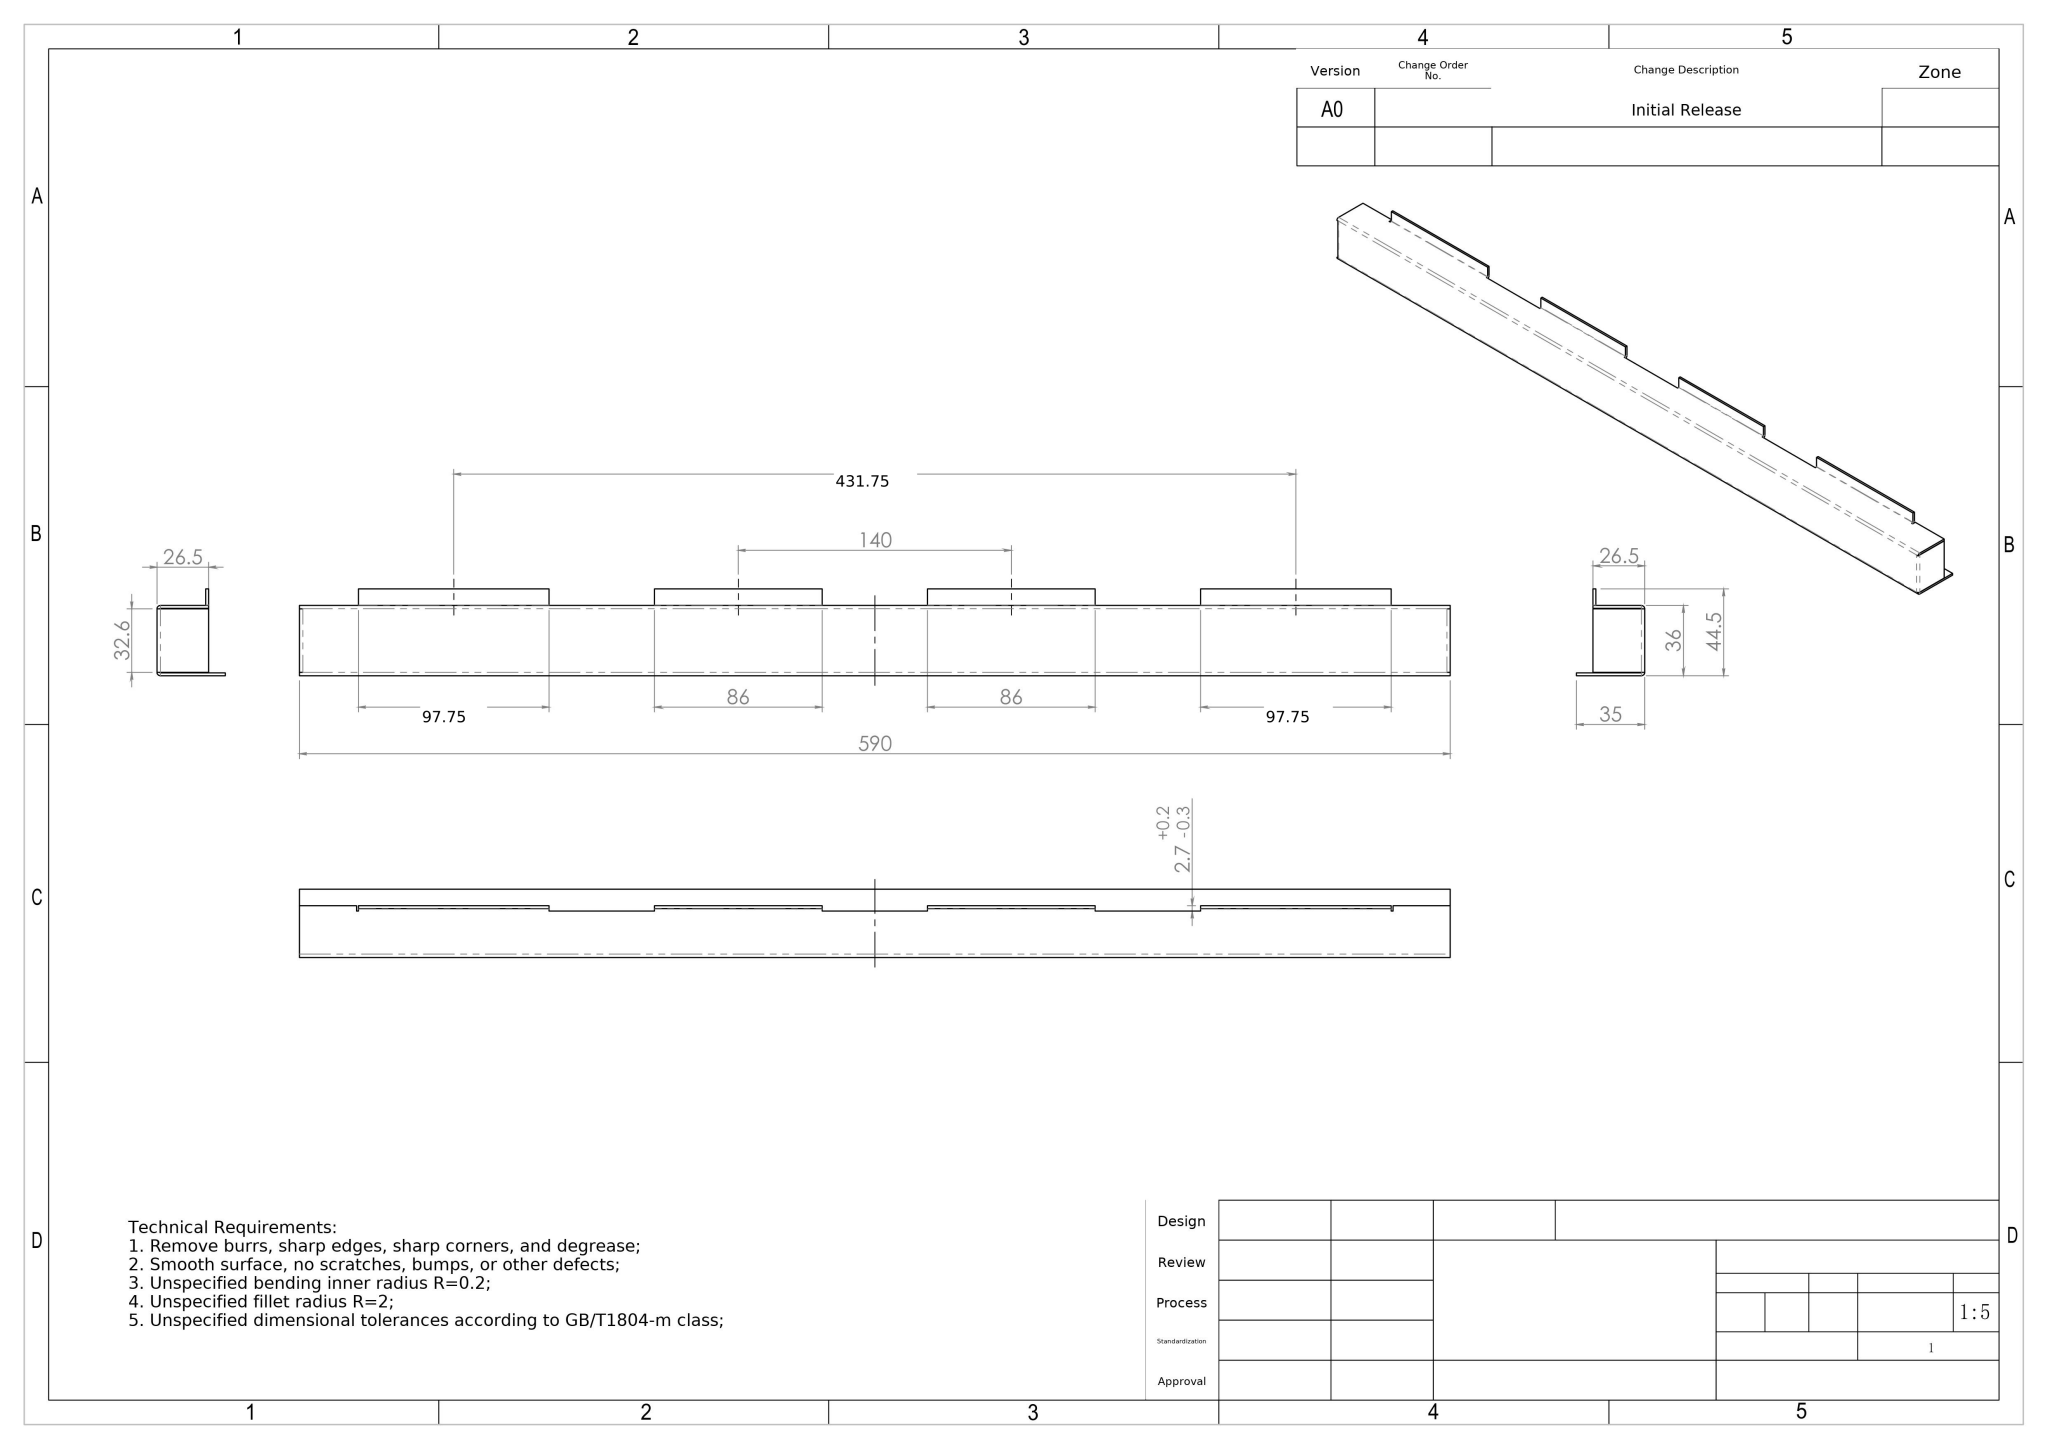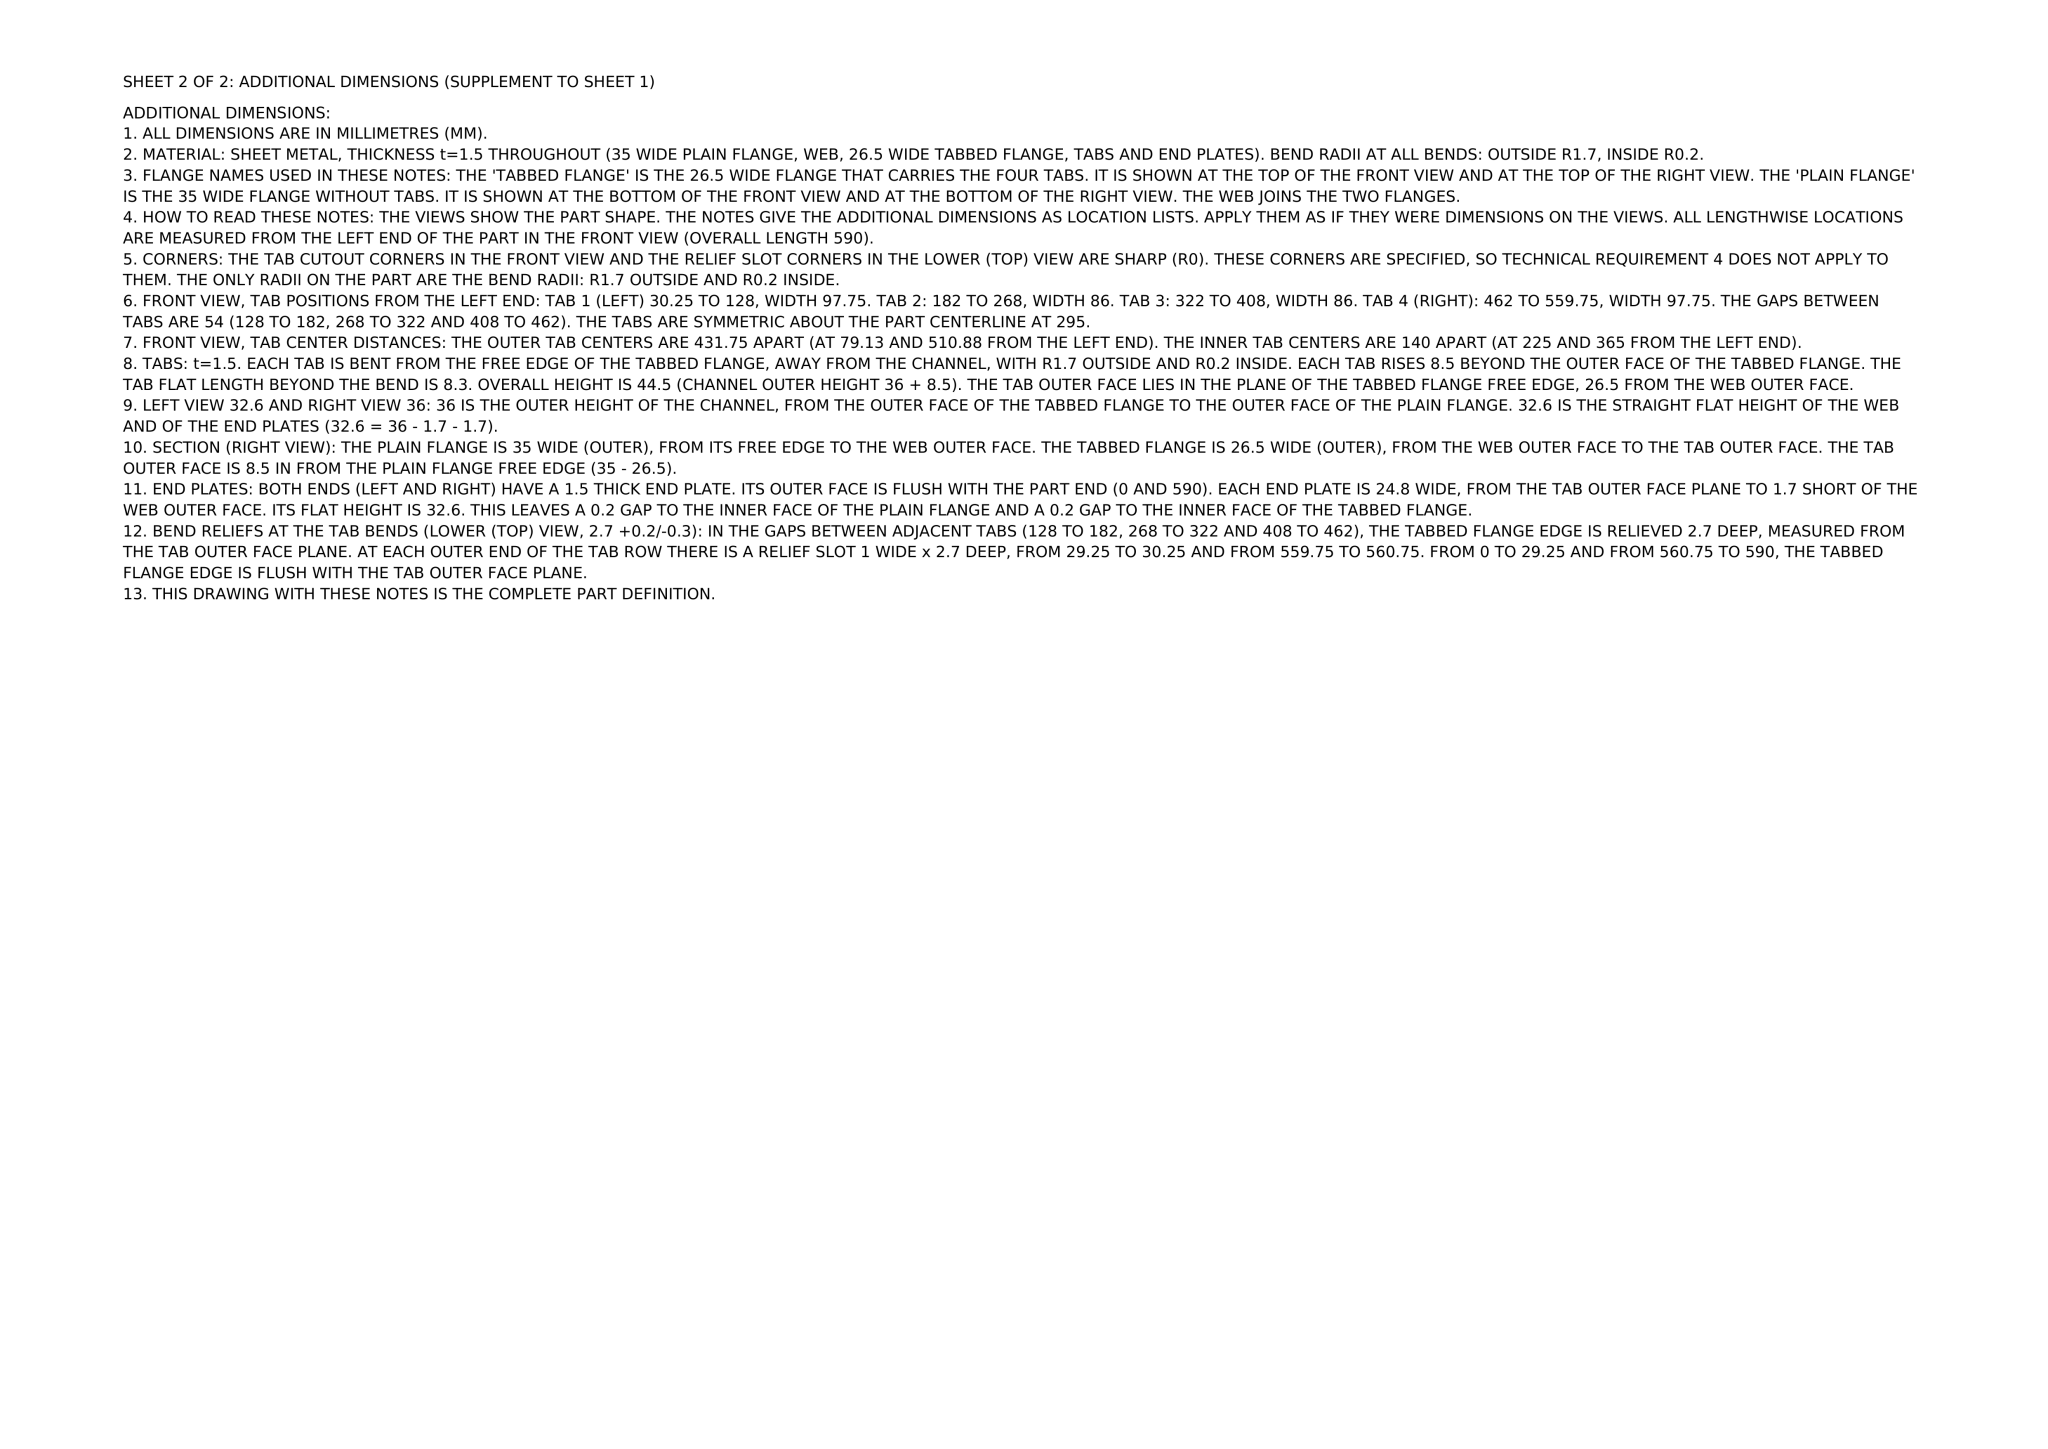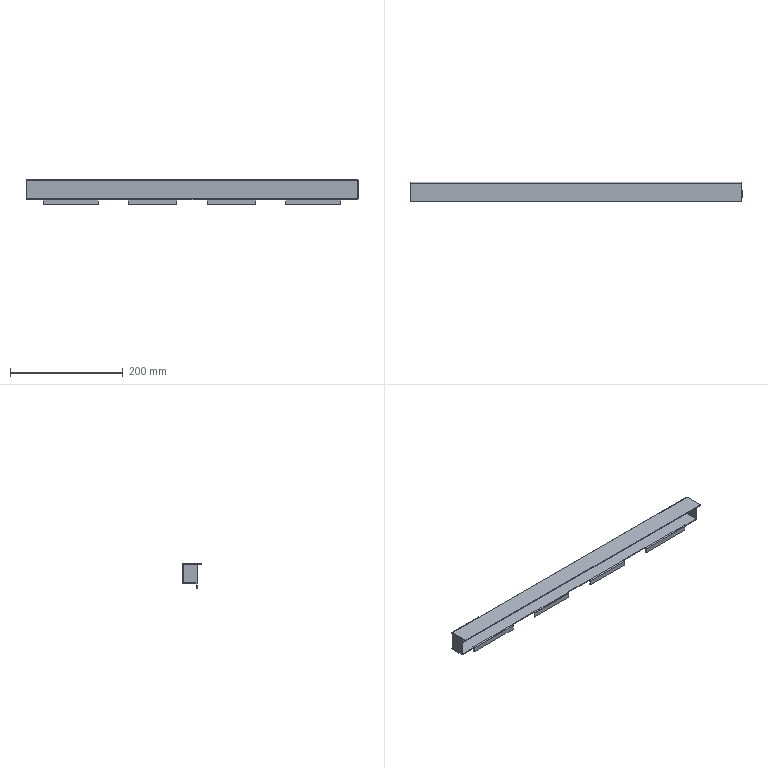Part | NX | mm | 1 solid | 94 faces | box 590 x 35 x 44.5 mm | volume 89113 mm3 | plane 78 | cylinder 16 | commonest cylinder face diameters 3.4 x8 0.4 x8